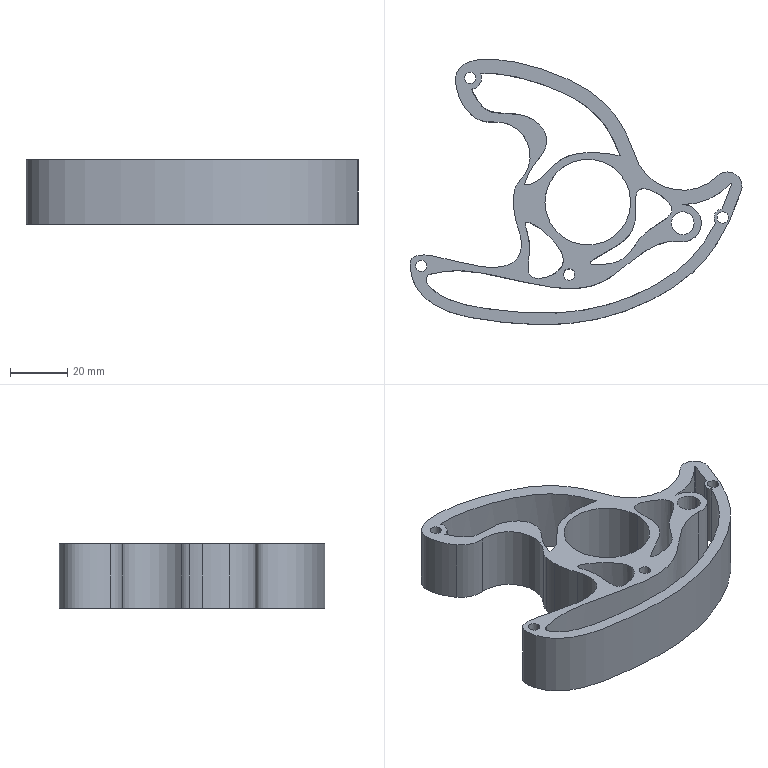Component | SolidWorks | ChainGuideSeat-1 | 1 solid | 43 faces | volume 54406 mm3 | cylinder 29 | spline 12 | plane 2 | commonest cylinder face diameters 4 x10 8 x3 6 x2 52 x2 30 x2 10 x2 35 x1 1.537 x1